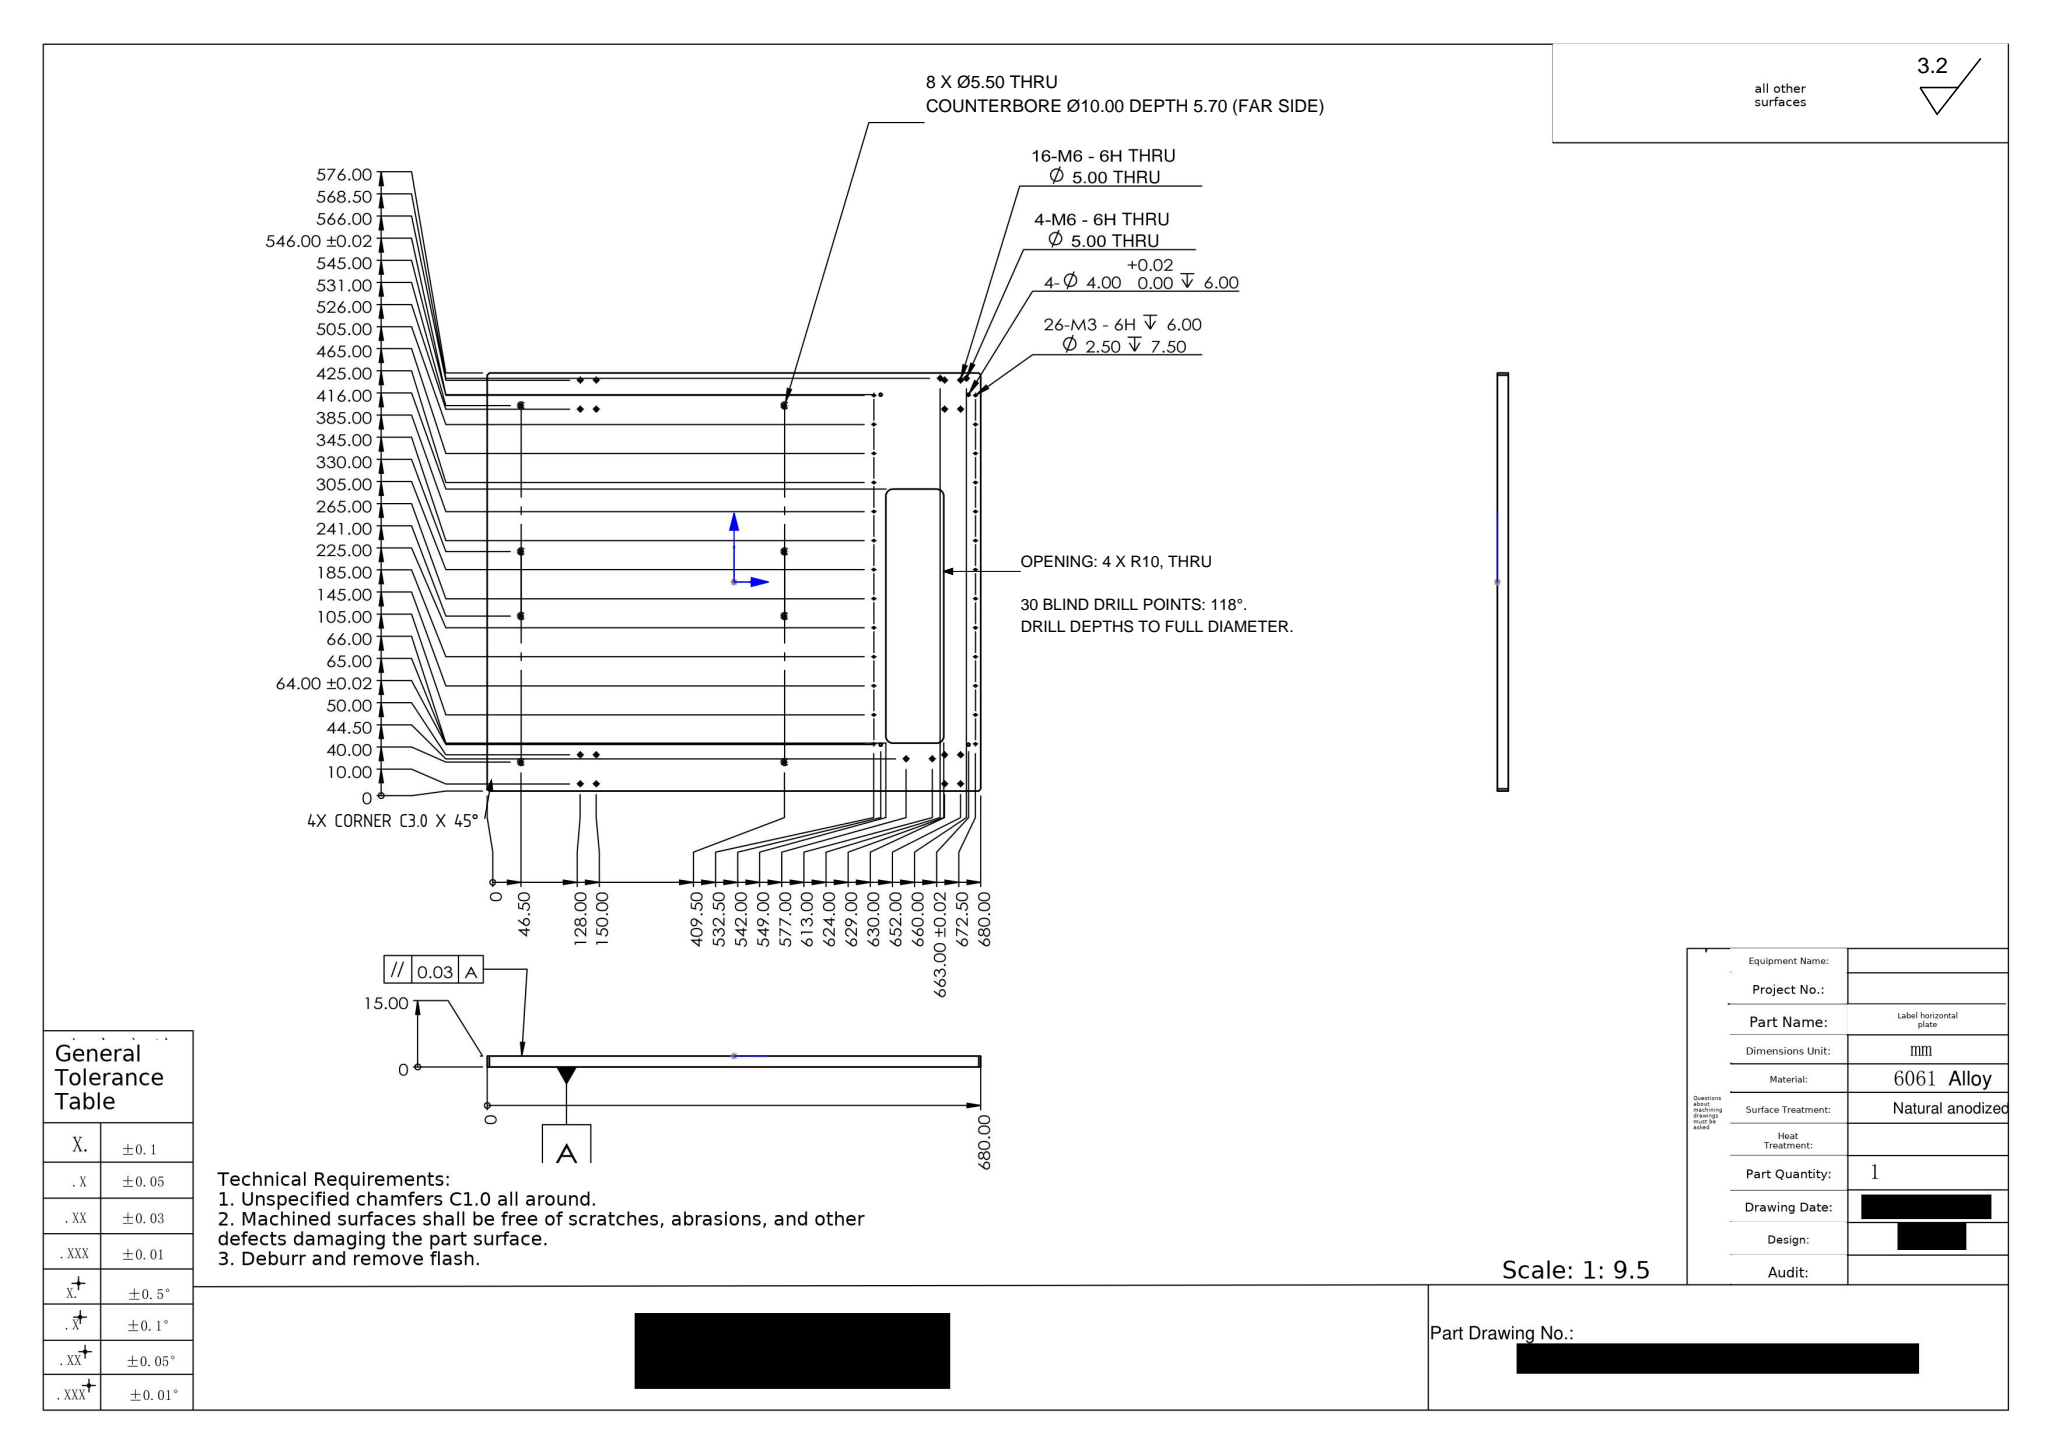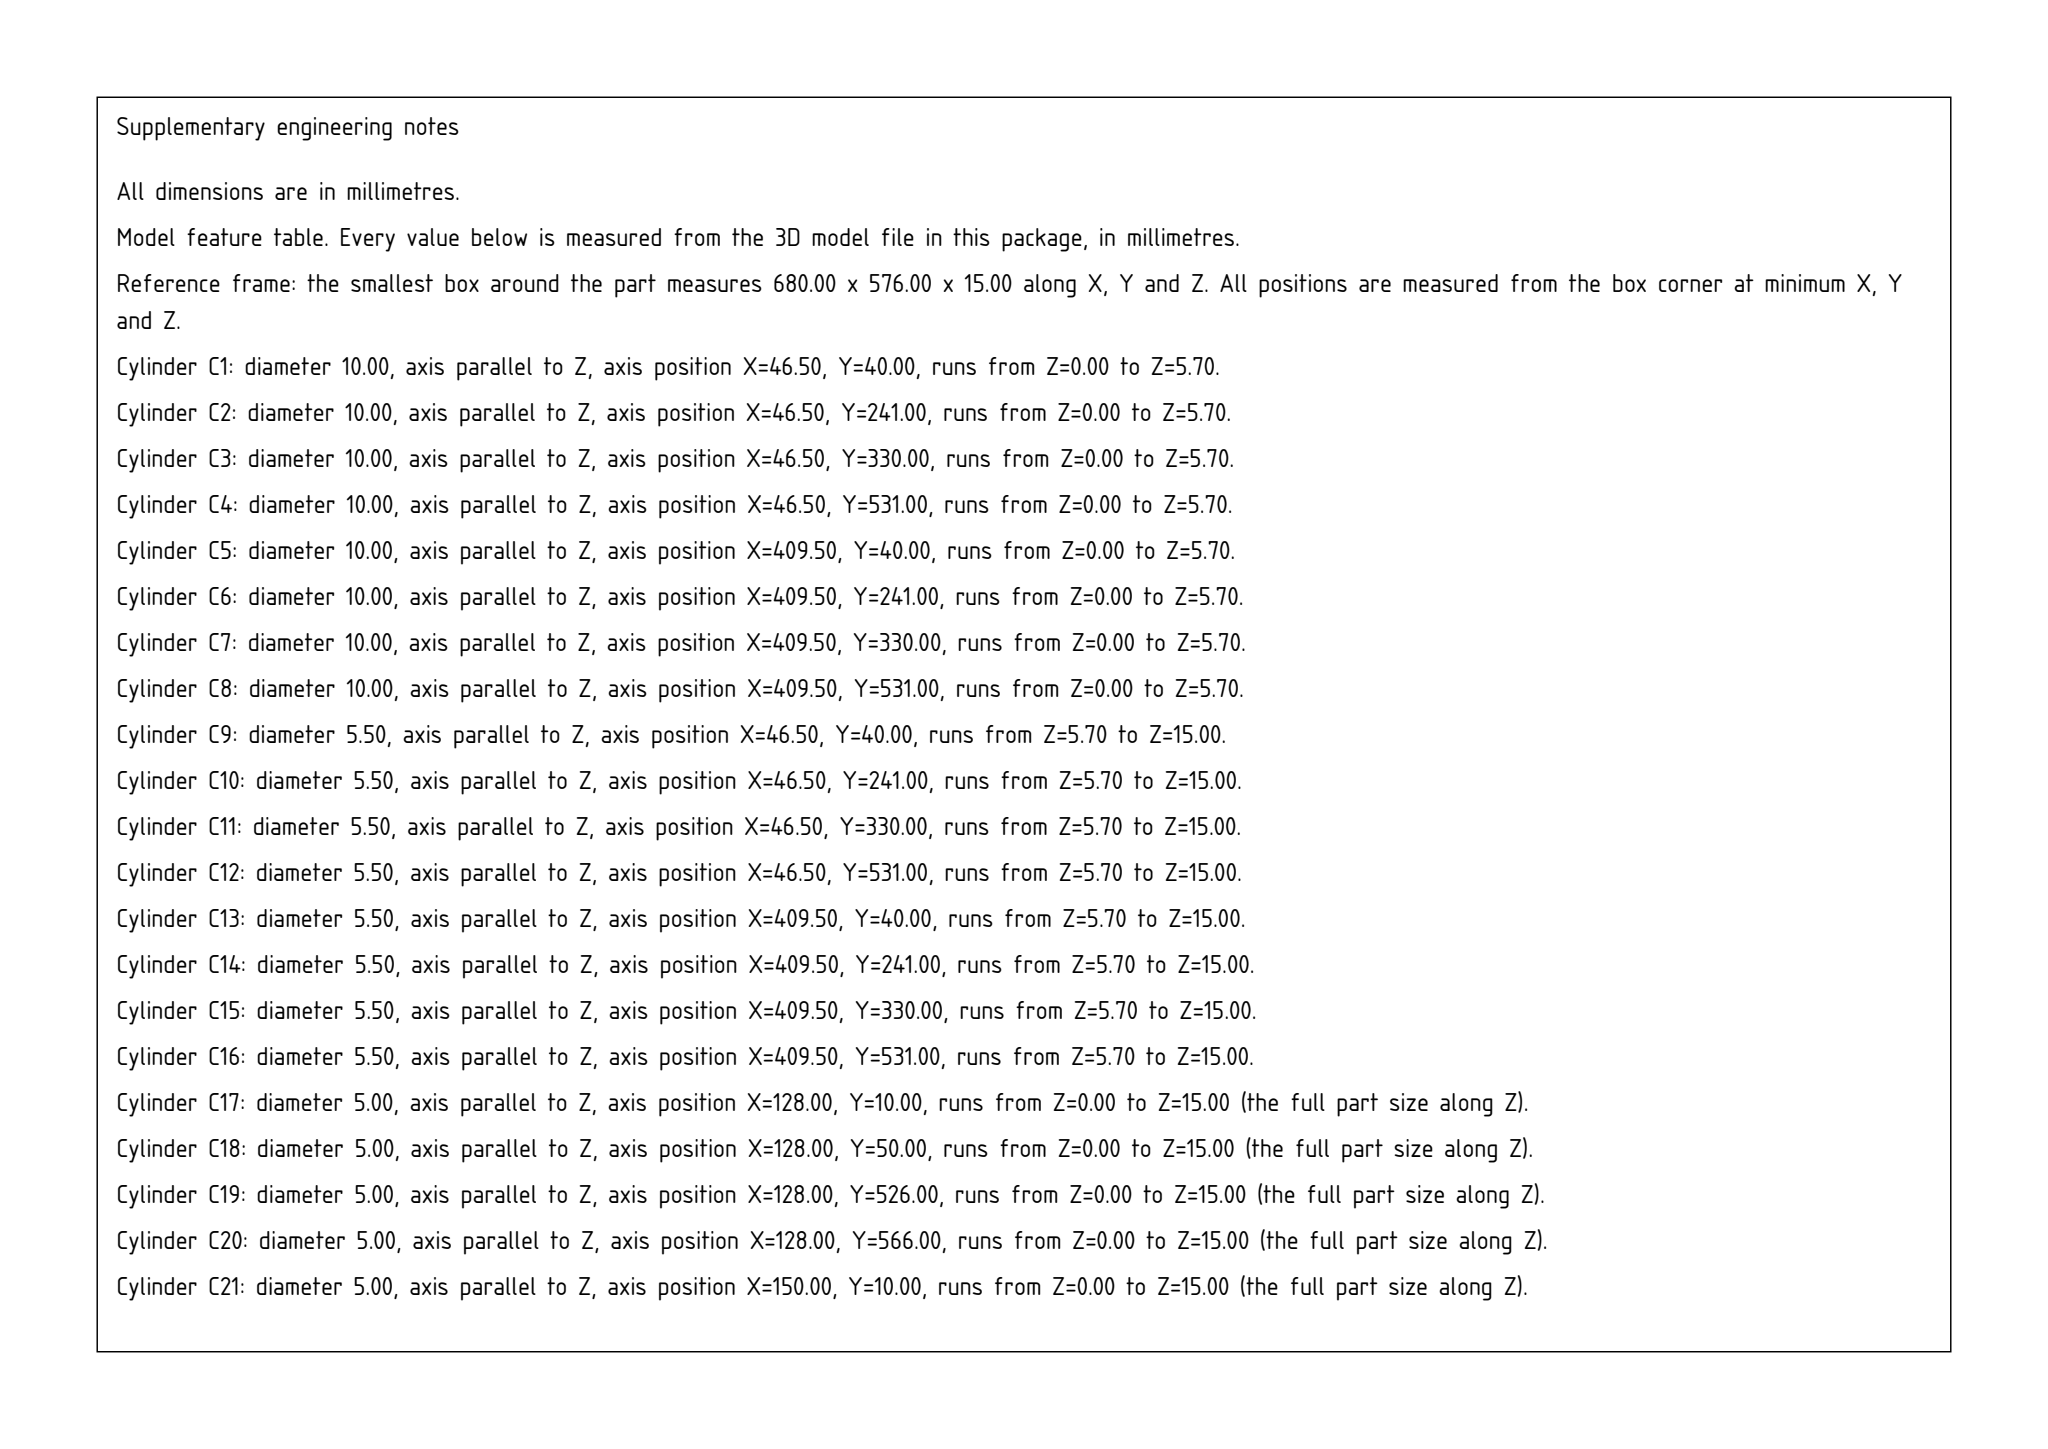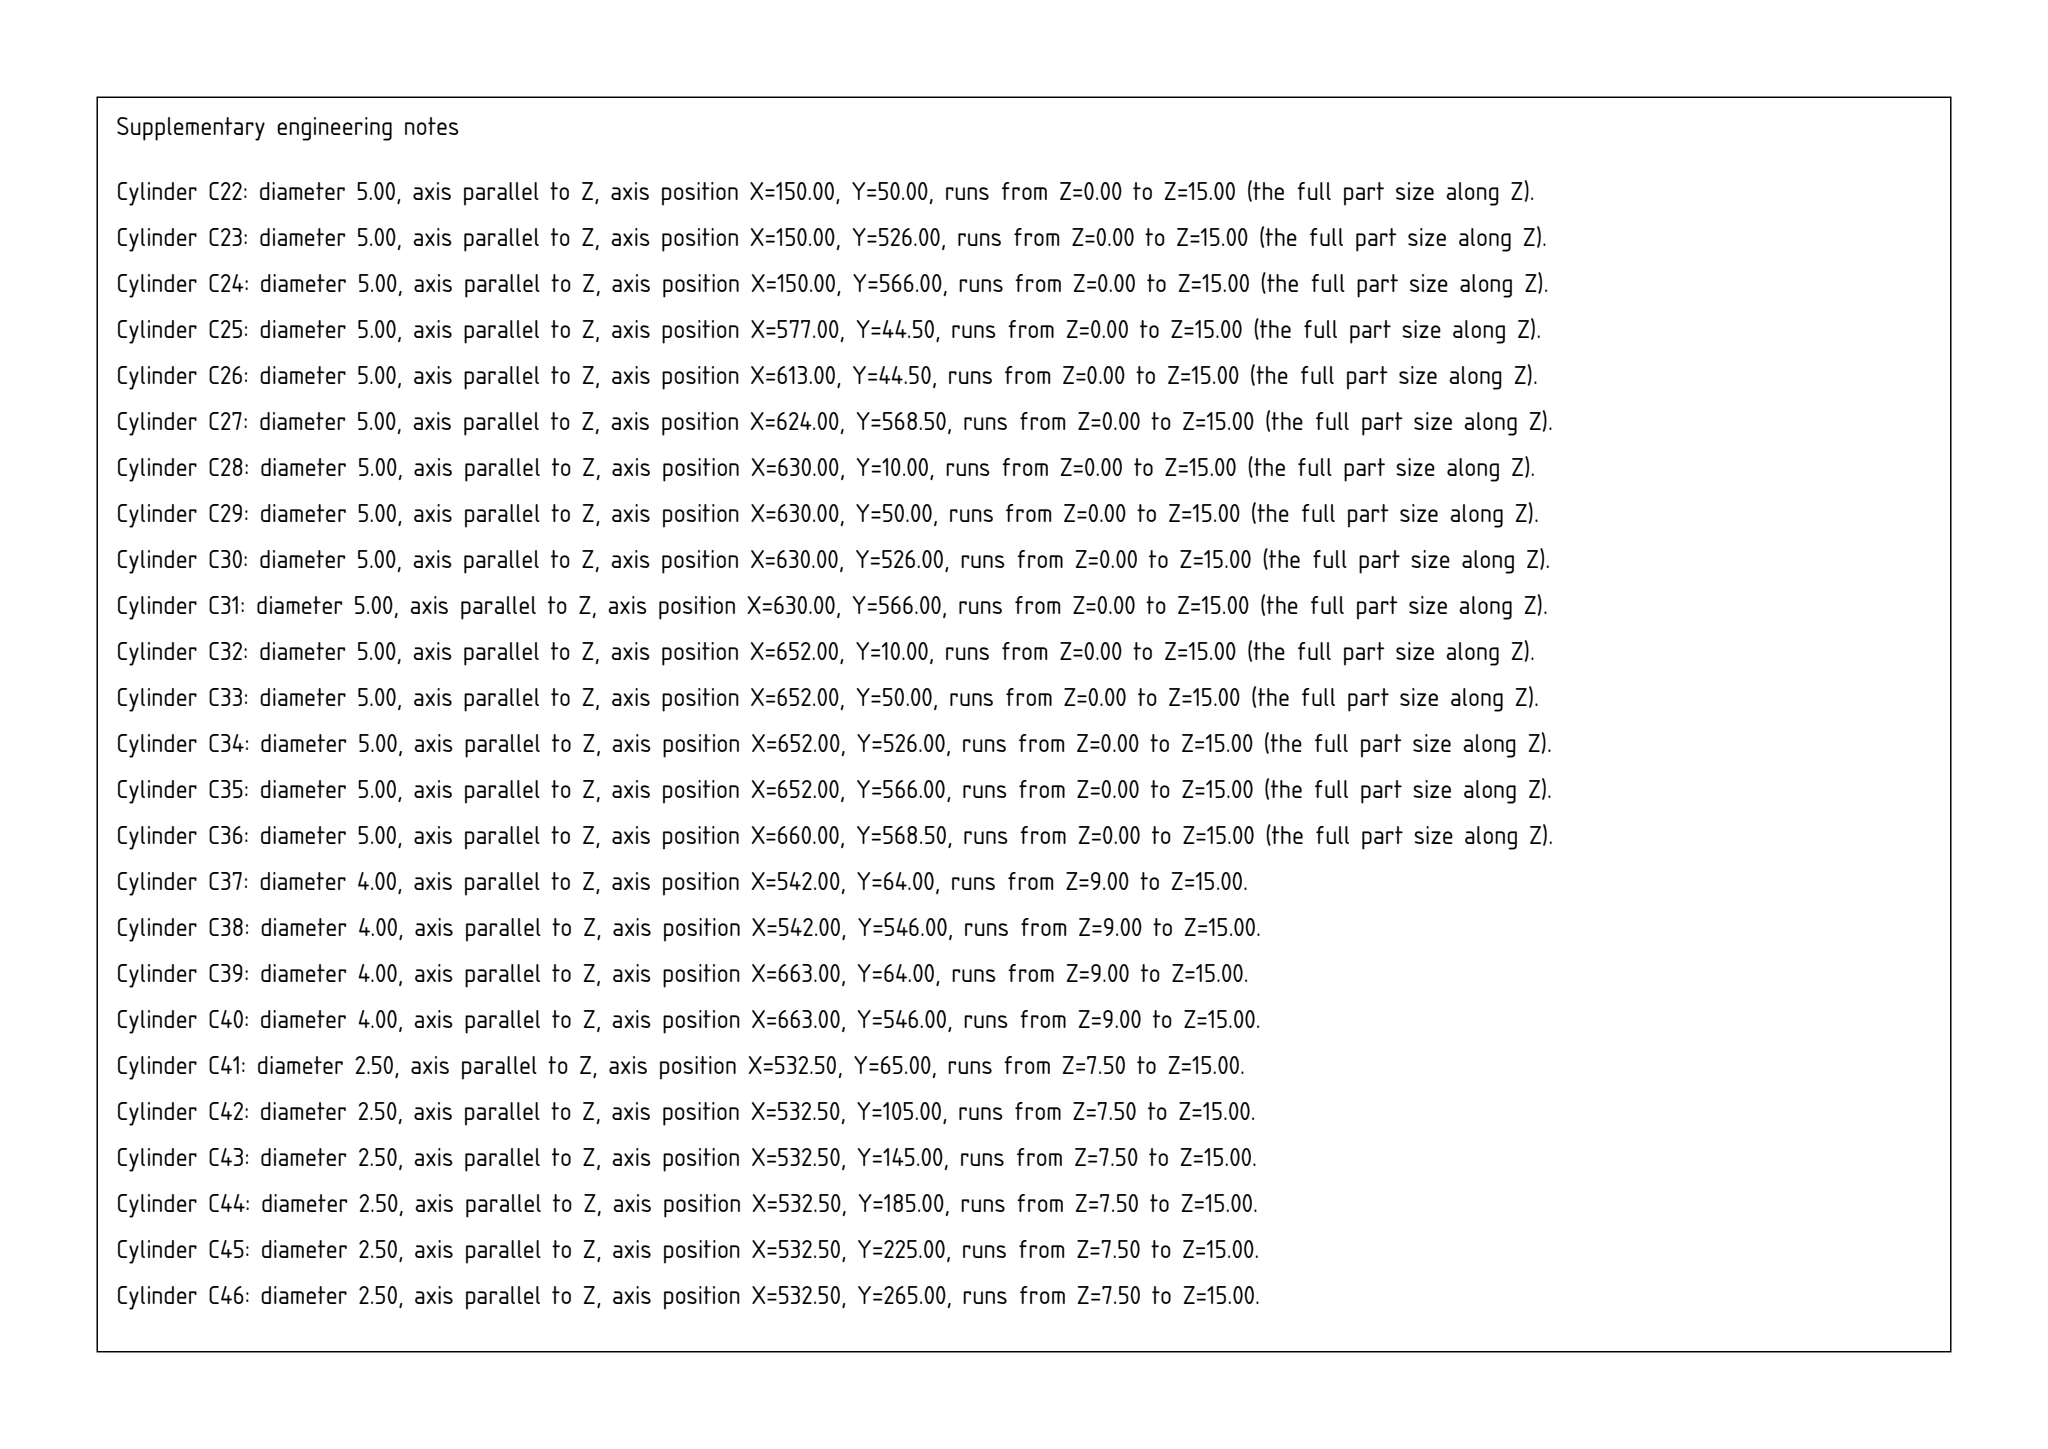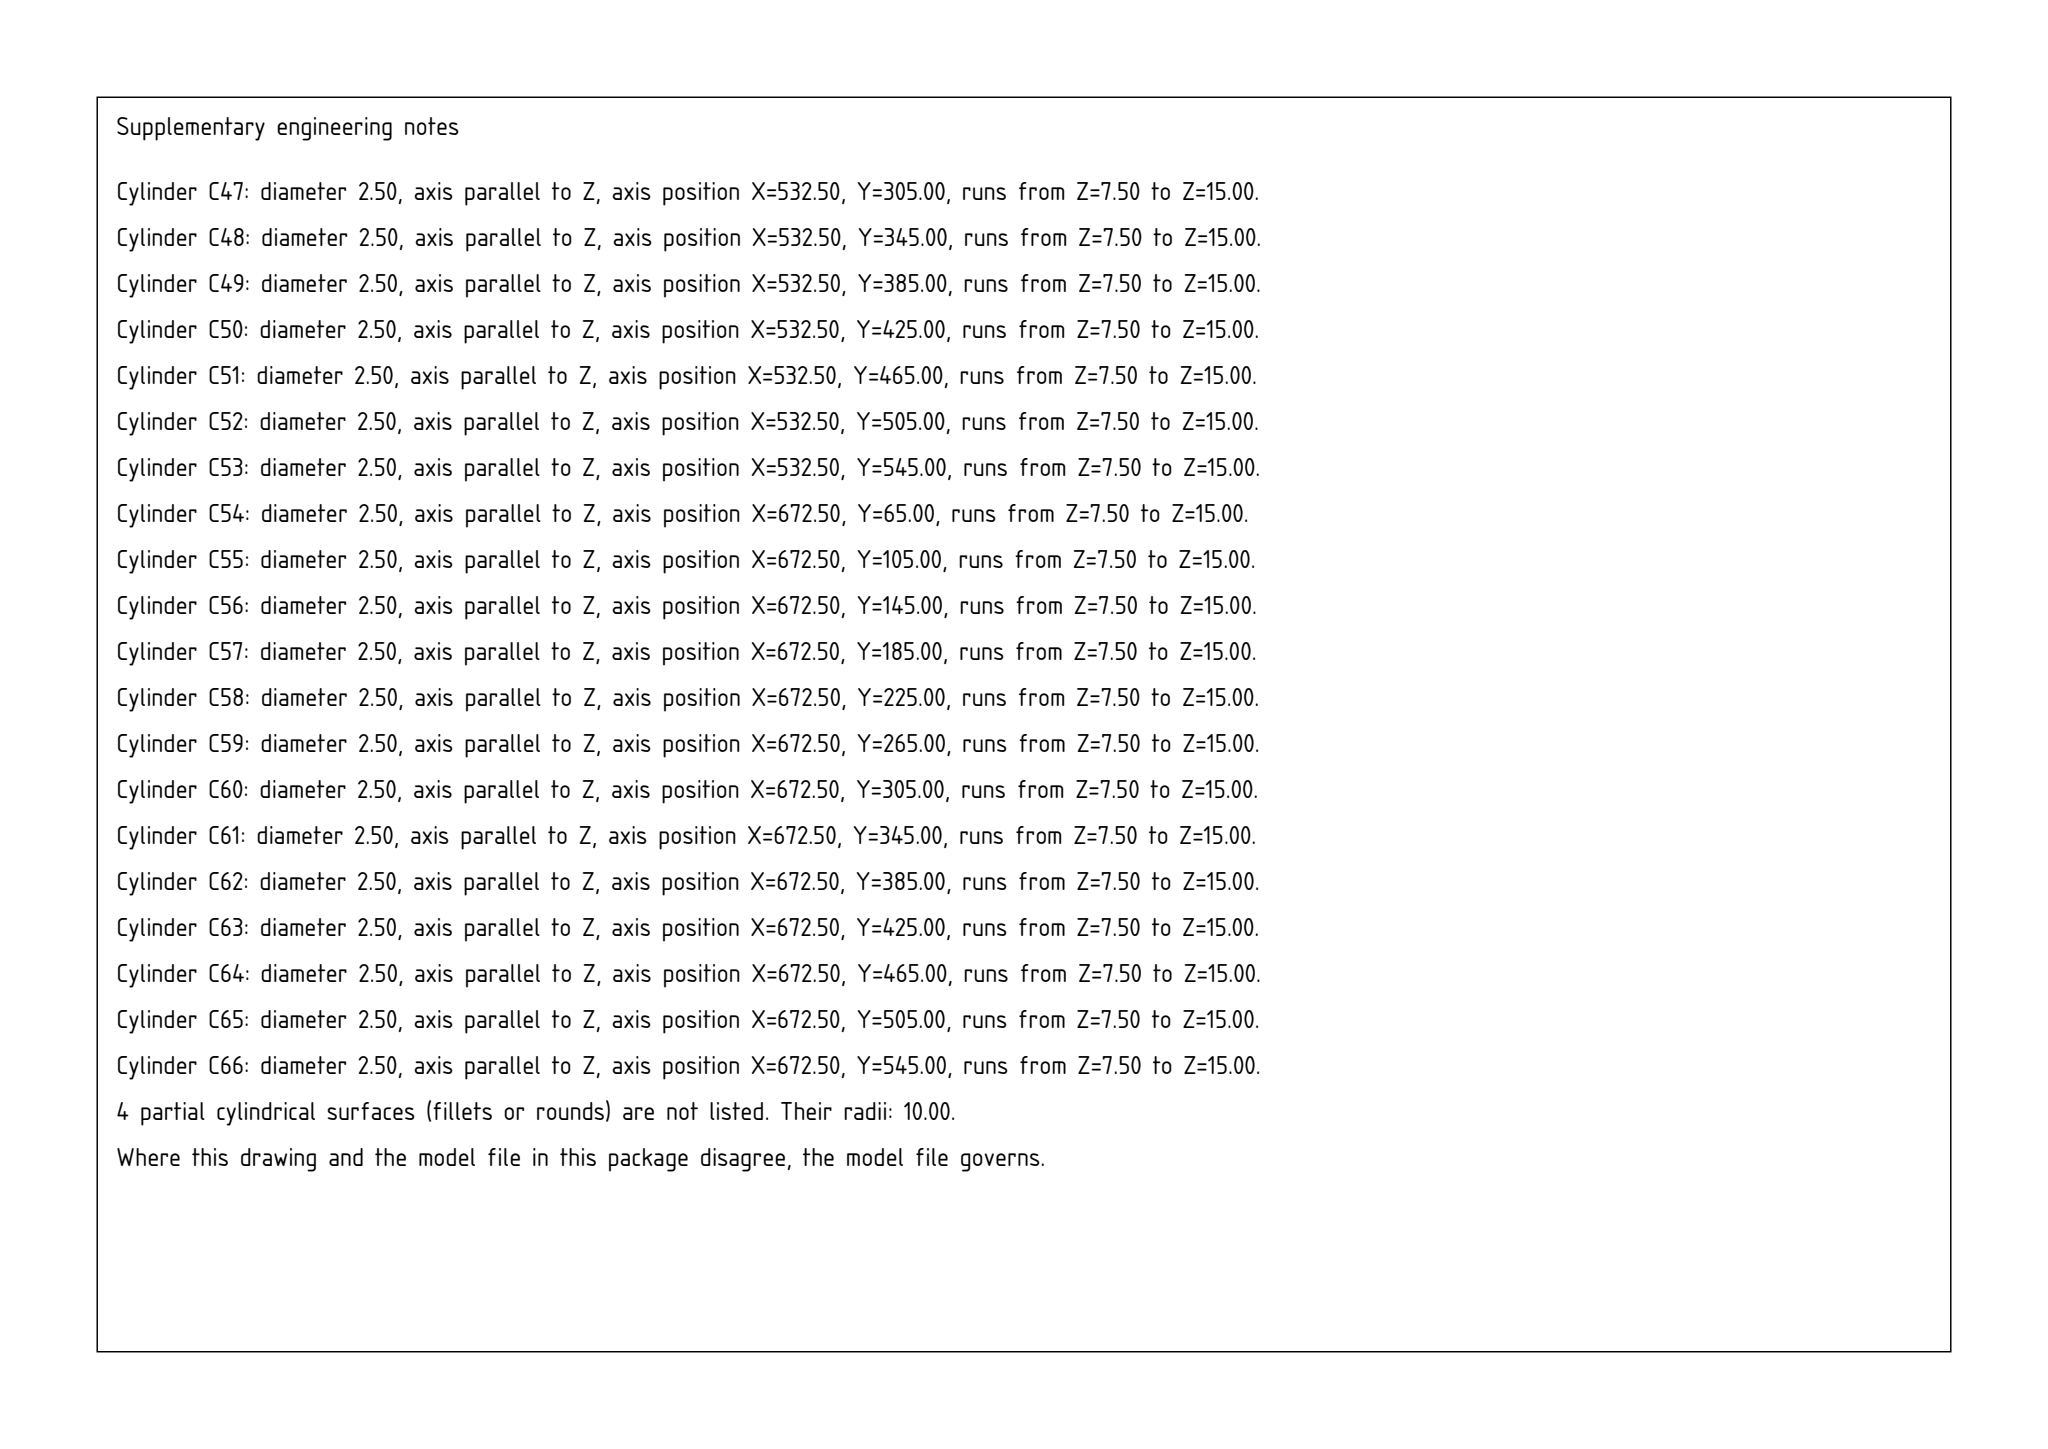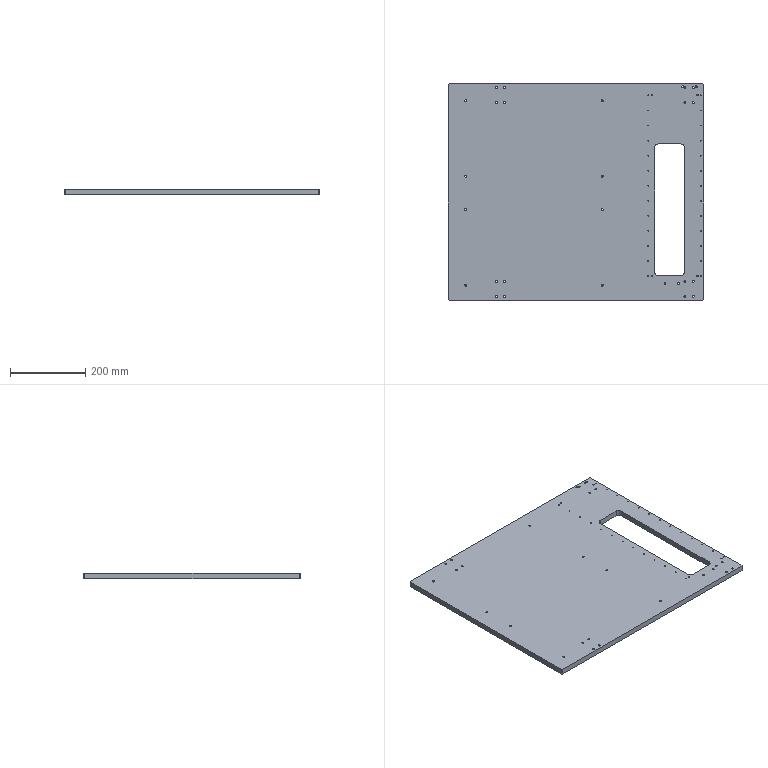Part | SolidWorks | mm | material 6061 Alloy | 1 solid | 218 faces | box 680 x 576 x 15 mm | volume 5443667 mm3 | cylinder 136 | cone 60 | plane 22 | commonest cylinder face diameters 2.5 x52 5 x40 10 x16 5.5 x16 4 x8 20 x4
Drawing notes:
4 X CORNER CHAMFER C3.0 X 45°, THRU 15 THK (NOT C1.0) | from the solid: inclined_planes: 4 faces 45°/45°, size [3.0,3.0,15.0] at corners (0,0),(0,573),(677,0),(677,573) of 680x576x15 bbox